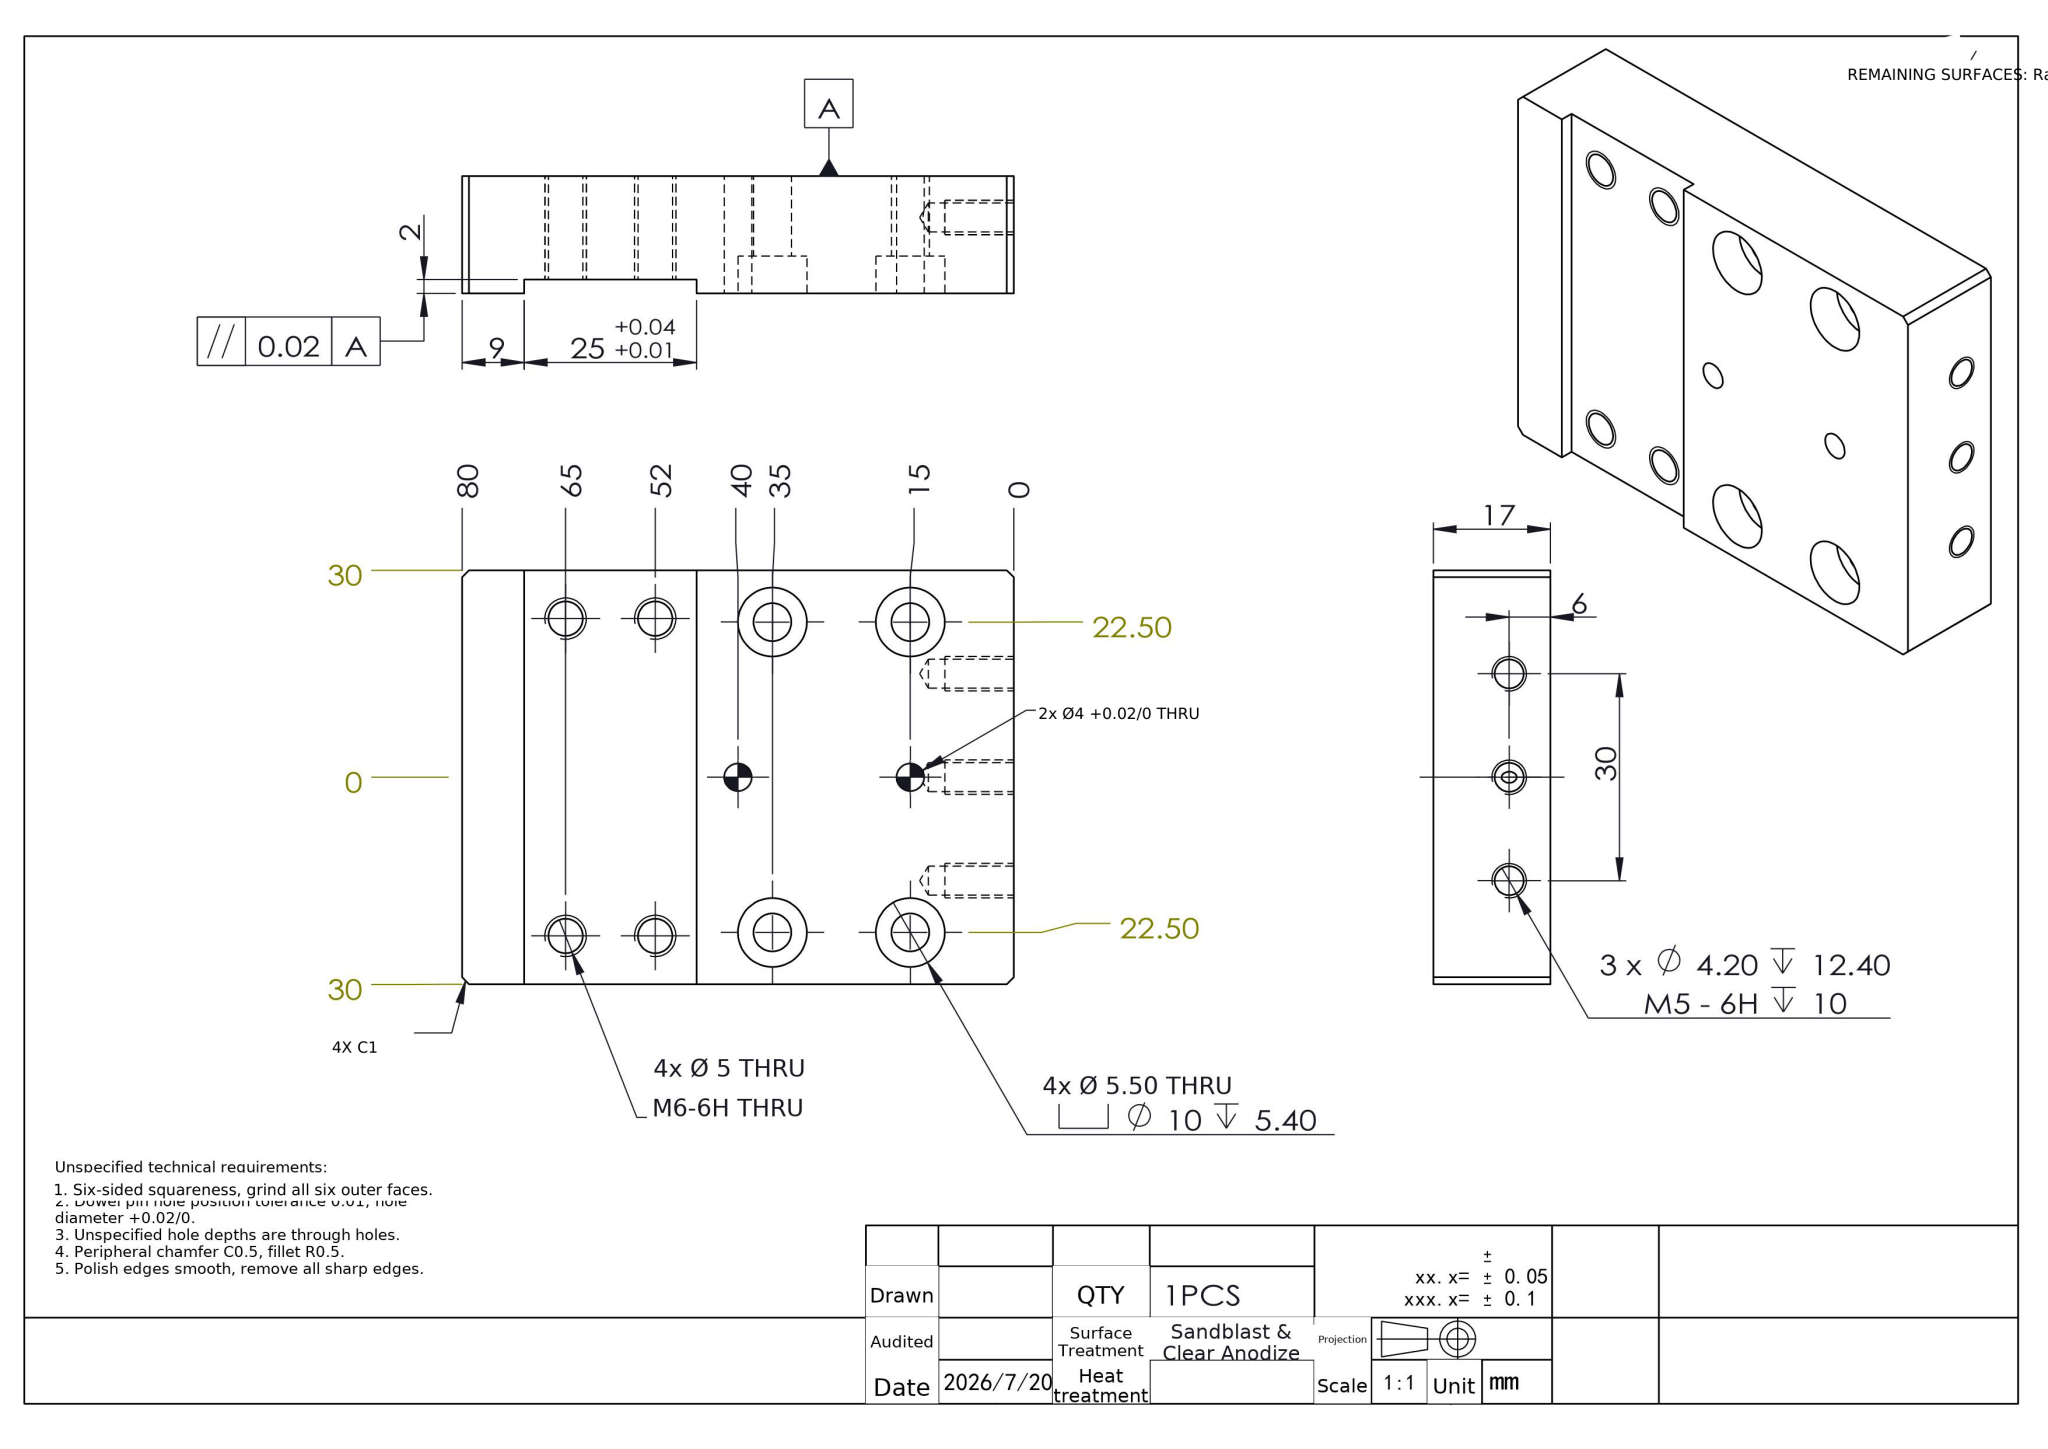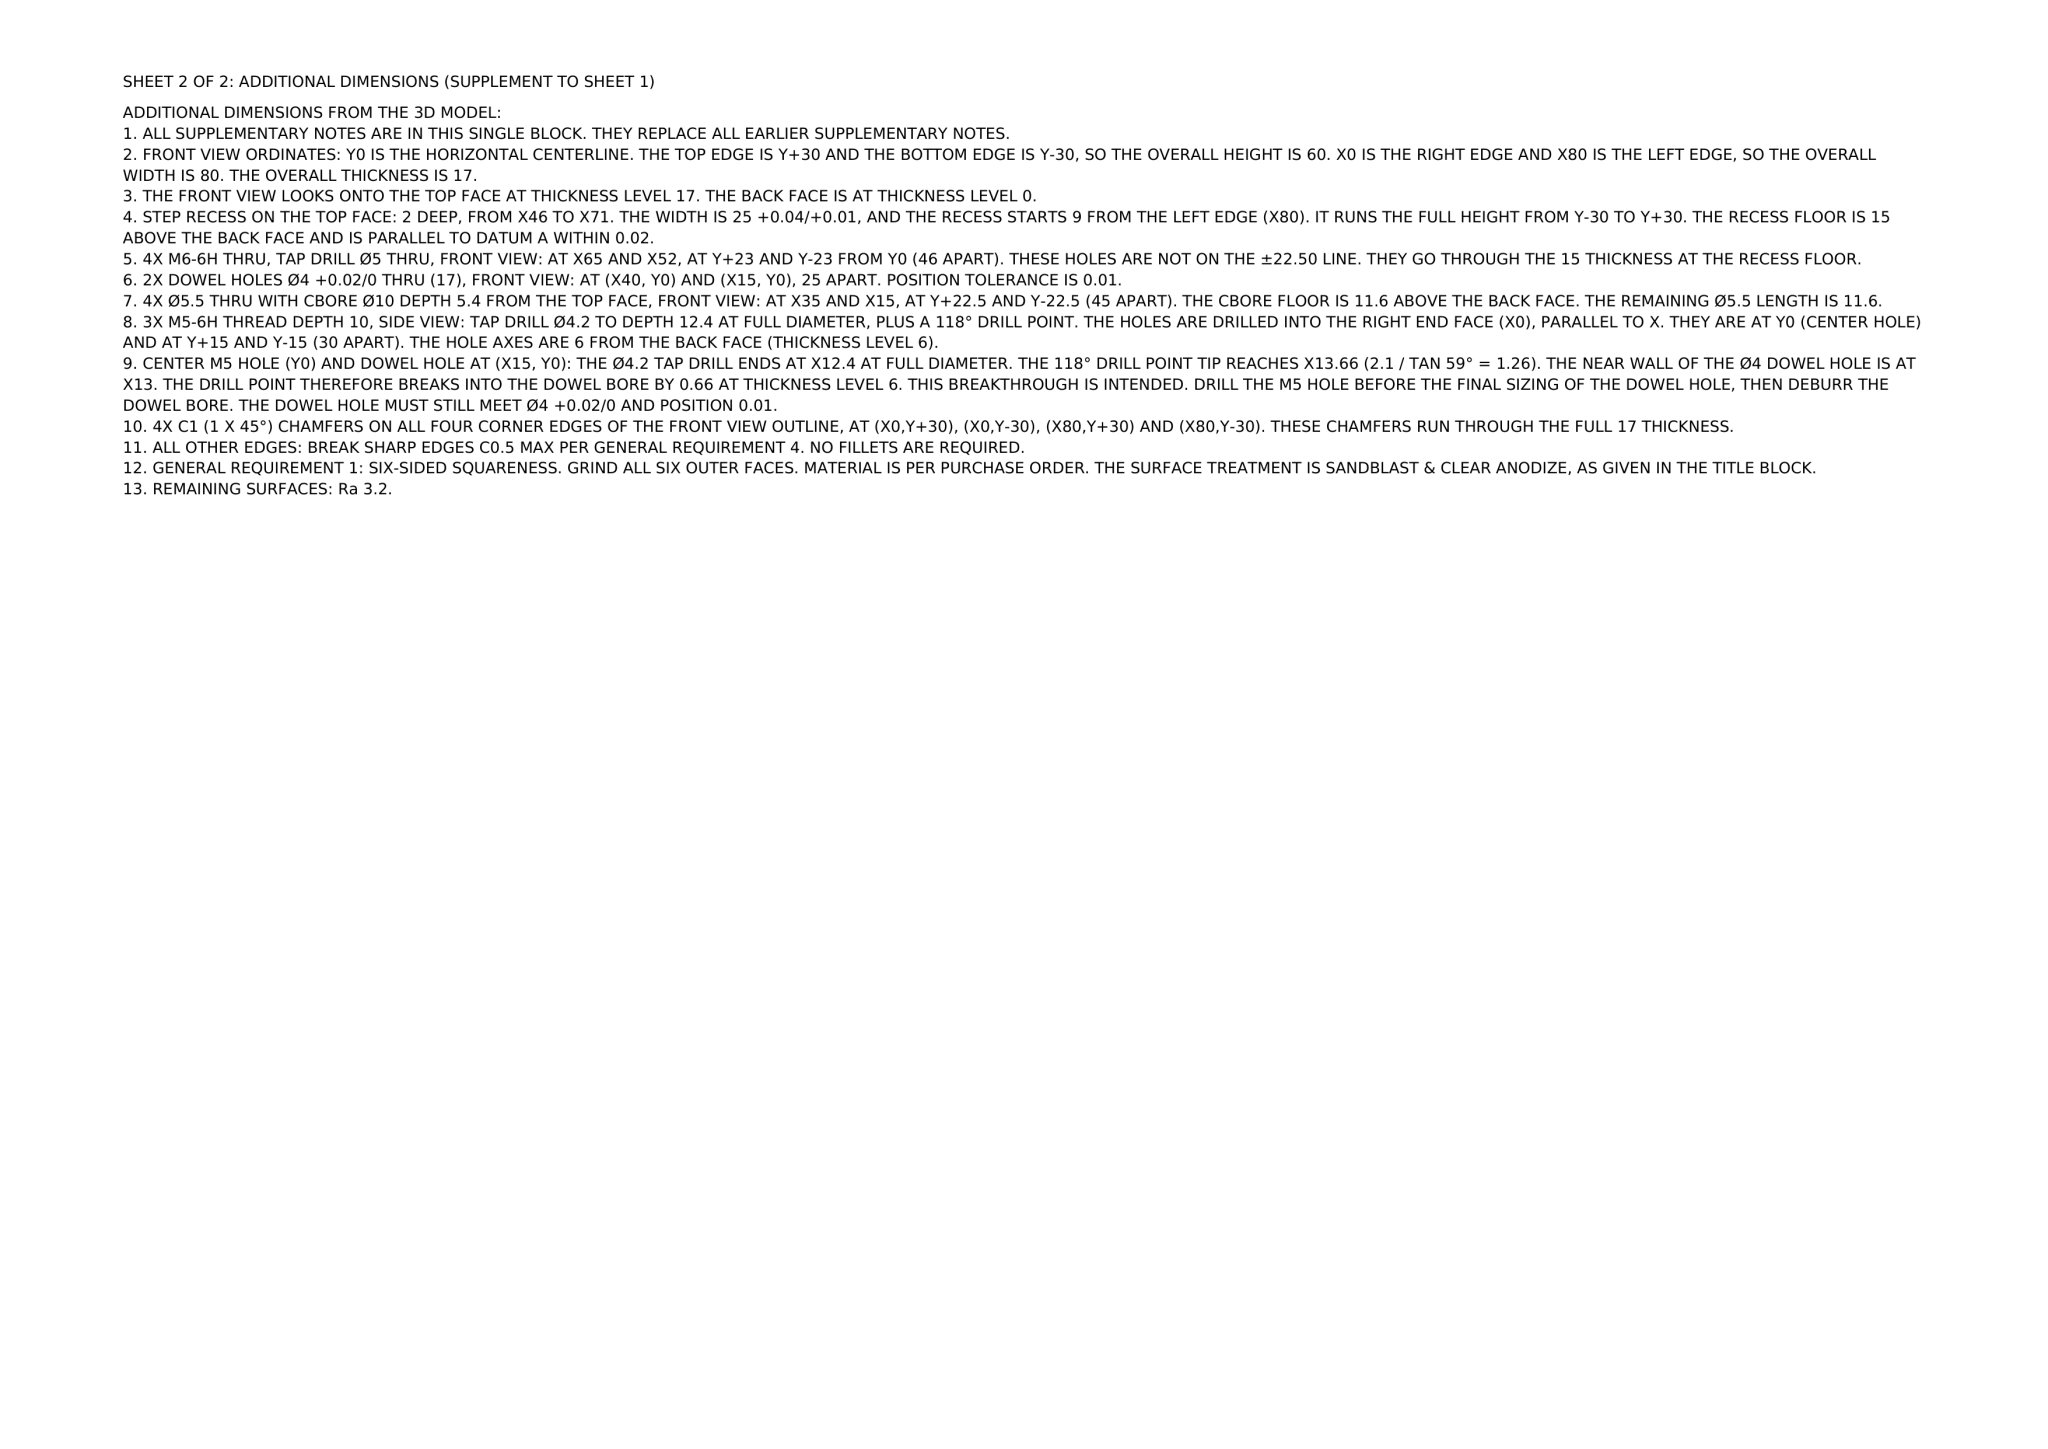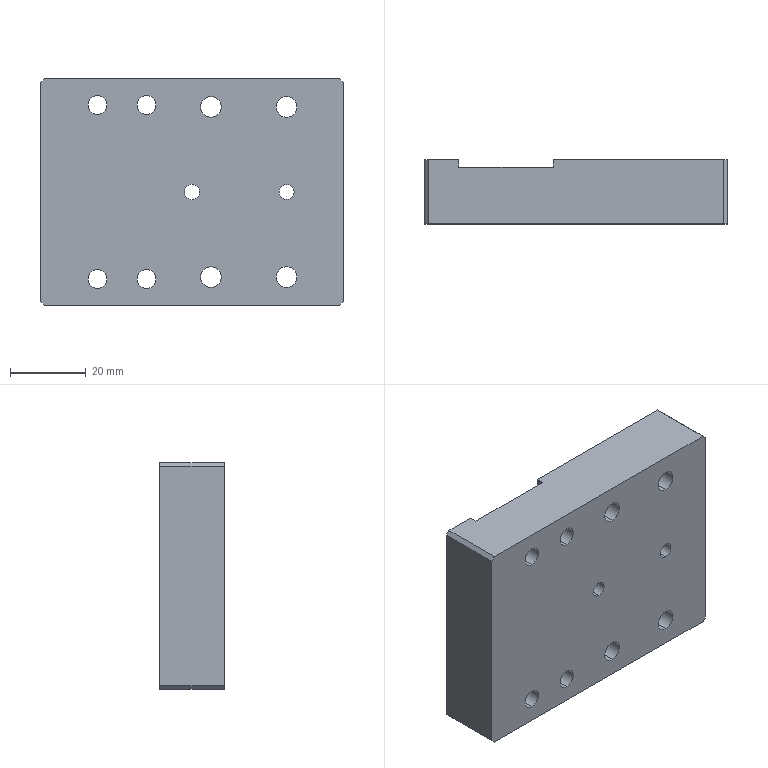Part | NX | mm | 1 solid | 58 faces | box 80 x 17 x 60 mm | volume 73630 mm3 | cylinder 34 | plane 18 | cone 6 | commonest cylinder face diameters 10 x8 5.5 x8 5 x8 4.2 x6 4 x4